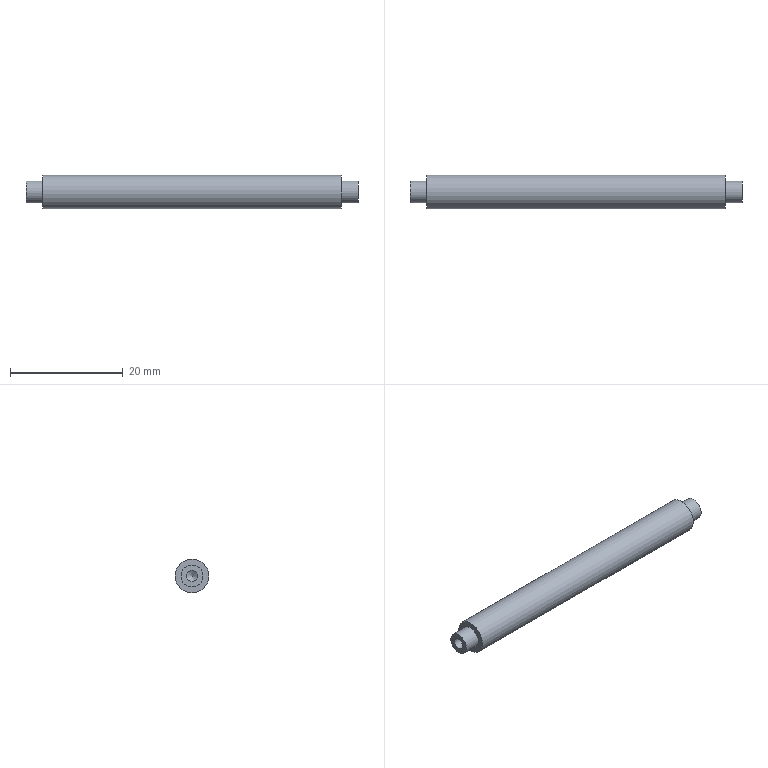Component | NX | SHAFT | 1 solid | 11 faces | box 59 x 6 x 6 mm | volume 1556 mm3 | cylinder 5 | plane 4 | cone 2 | commonest cylinder face diameters 3.9 x2 2 x2 6 x1
STEP:
#1=CARTESIAN_POINT('',(0.,0.,0.));
#2=DIRECTION('',(0.,0.,1.));
#3=DIRECTION('',(1.,0.,0.));
#4=AXIS2_PLACEMENT_3D('',#1,#2,#3);
#5=CARTESIAN_POINT('',(12.144,27.69,-75.915));
#6=VERTEX_POINT('',#5);
#7=CARTESIAN_POINT('',(12.144,27.69,-72.915));
#8=DIRECTION('',(1.,0.,0.));
#9=DIRECTION('',(0.,0.,-1.));
#10=AXIS2_PLACEMENT_3D('',#7,#8,#9);
#11=CIRCLE('',#10,3.);
#12=CARTESIAN_POINT('',(12.144,27.69,-72.915));
#13=DIRECTION('',(-1.,0.,0.));
#14=DIRECTION('',(0.,0.,1.));
#15=AXIS2_PLACEMENT_3D('',#12,#13,#14);
#16=CYLINDRICAL_SURFACE('',#15,3.);
#17=CARTESIAN_POINT('',(9.425,0.));
#18=DIRECTION('',(-1.,0.));
#19=VECTOR('',#18,1.);
#20=LINE('',#17,#19);
#21=(GEOMETRIC_REPRESENTATION_CONTEXT(2)PARAMETRIC_REPRESENTATION_CONTEXT()REPRESENTATION_CONTEXT('',''));
#22=DEFINITIONAL_REPRESENTATION('',(#20),#21);
#23=PCURVE('',#16,#22);
#24=CARTESIAN_POINT('',(12.144,27.69,-72.915));
#25=DIRECTION('',(1.,0.,0.));
#26=DIRECTION('',(0.,0.,-1.));
#27=AXIS2_PLACEMENT_3D('',#24,#25,#26);
#28=PLANE('',#27);
#29=CARTESIAN_POINT('',(0.,0.));
#30=DIRECTION('',(1.,0.));
#31=AXIS2_PLACEMENT_2D('',#29,#30);
#32=CIRCLE('',#31,3.);
#33=(GEOMETRIC_REPRESENTATION_CONTEXT(2)PARAMETRIC_REPRESENTATION_CONTEXT()REPRESENTATION_CONTEXT('',''));
#34=DEFINITIONAL_REPRESENTATION('',(#32),#33);
#35=PCURVE('',#28,#34);
#36=SURFACE_CURVE('',#11,(#23,#35),.PCURVE_S1.);
#37=EDGE_CURVE('',#6,#6,#36,.T.);
#38=ORIENTED_EDGE('',*,*,#37,.F.);
#39=CARTESIAN_POINT('',(-40.856,27.69,-75.915));
#40=VERTEX_POINT('',#39);
#41=CARTESIAN_POINT('',(12.144,27.69,-75.915));
#42=CARTESIAN_POINT('',(-40.856,27.69,-75.915));
#43=B_SPLINE_CURVE_WITH_KNOTS('',1,(#41,#42),.UNSPECIFIED.,.F.,.F.,(2,2),(0.,53.),.PIECEWISE_BEZIER_KNOTS.);
#44=CARTESIAN_POINT('',(9.425,0.));
#45=DIRECTION('',(0.,1.));
#46=VECTOR('',#45,1.);
#47=LINE('',#44,#46);
#48=(GEOMETRIC_REPRESENTATION_CONTEXT(2)PARAMETRIC_REPRESENTATION_CONTEXT()REPRESENTATION_CONTEXT('',''));
#49=DEFINITIONAL_REPRESENTATION('',(#47),#48);
#50=PCURVE('',#16,#49);
#51=CARTESIAN_POINT('',(3.142,0.));
#52=DIRECTION('',(0.,1.));
#53=VECTOR('',#52,1.);
#54=LINE('',#51,#53);
#55=(GEOMETRIC_REPRESENTATION_CONTEXT(2)PARAMETRIC_REPRESENTATION_CONTEXT()REPRESENTATION_CONTEXT('',''));
#56=DEFINITIONAL_REPRESENTATION('',(#54),#55);
#57=PCURVE('',#16,#56);
#58=SEAM_CURVE('',#43,(#50,#57),.PCURVE_S1.);
#59=EDGE_CURVE('',#6,#40,#58,.T.);
#60=ORIENTED_EDGE('',*,*,#59,.T.);
#61=CARTESIAN_POINT('',(-40.856,27.69,-72.915));
#62=DIRECTION('',(1.,0.,0.));
#63=DIRECTION('',(0.,0.,-1.));
#64=AXIS2_PLACEMENT_3D('',#61,#62,#63);
#65=CIRCLE('',#64,3.);
#66=CARTESIAN_POINT('',(9.425,53.));
#67=DIRECTION('',(-1.,0.));
#68=VECTOR('',#67,1.);
#69=LINE('',#66,#68);
#70=(GEOMETRIC_REPRESENTATION_CONTEXT(2)PARAMETRIC_REPRESENTATION_CONTEXT()REPRESENTATION_CONTEXT('',''));
#71=DEFINITIONAL_REPRESENTATION('',(#69),#70);
#72=PCURVE('',#16,#71);
#73=CARTESIAN_POINT('',(-40.856,27.69,-72.915));
#74=DIRECTION('',(1.,0.,0.));
#75=DIRECTION('',(0.,0.,-1.));
#76=AXIS2_PLACEMENT_3D('',#73,#74,#75);
#77=PLANE('',#76);
#78=CARTESIAN_POINT('',(0.,0.));
#79=DIRECTION('',(1.,0.));
#80=AXIS2_PLACEMENT_2D('',#78,#79);
#81=CIRCLE('',#80,3.);
#82=(GEOMETRIC_REPRESENTATION_CONTEXT(2)PARAMETRIC_REPRESENTATION_CONTEXT()REPRESENTATION_CONTEXT('',''));
#83=DEFINITIONAL_REPRESENTATION('',(#81),#82);
#84=PCURVE('',#77,#83);
#85=SURFACE_CURVE('',#65,(#72,#84),.PCURVE_S1.);
#86=EDGE_CURVE('',#40,#40,#85,.T.);
#87=ORIENTED_EDGE('',*,*,#86,.T.);
#88=ORIENTED_EDGE('',*,*,#59,.F.);
#89=EDGE_LOOP('',(#38,#60,#87,#88));
#90=FACE_BOUND('',#89,.T.);
#91=ADVANCED_FACE('',(#90),#16,.T.);
#92=CARTESIAN_POINT('',(12.144,27.69,-74.865));
#93=VERTEX_POINT('',#92);
#94=CARTESIAN_POINT('',(12.144,27.69,-72.915));
#95=DIRECTION('',(1.,0.,0.));
#96=DIRECTION('',(0.,0.,-1.));
#97=AXIS2_PLACEMENT_3D('',#94,#95,#96);
#98=CIRCLE('',#97,1.95);
#99=CARTESIAN_POINT('',(0.,0.));
#100=DIRECTION('',(1.,0.));
#101=AXIS2_PLACEMENT_2D('',#99,#100);
#102=CIRCLE('',#101,1.95);
#103=(GEOMETRIC_REPRESENTATION_CONTEXT(2)PARAMETRIC_REPRESENTATION_CONTEXT()REPRESENTATION_CONTEXT('',''));
#104=DEFINITIONAL_REPRESENTATION('',(#102),#103);
#105=PCURVE('',#28,#104);
#106=CARTESIAN_POINT('',(15.144,27.69,-72.915));
#107=DIRECTION('',(-1.,0.,0.));
#108=DIRECTION('',(0.,0.,1.));
#109=AXIS2_PLACEMENT_3D('',#106,#107,#108);
#110=CYLINDRICAL_SURFACE('',#109,1.95);
#111=CARTESIAN_POINT('',(9.425,3.));
#112=DIRECTION('',(-1.,0.));
#113=VECTOR('',#112,1.);
#114=LINE('',#111,#113);
#115=(GEOMETRIC_REPRESENTATION_CONTEXT(2)PARAMETRIC_REPRESENTATION_CONTEXT()REPRESENTATION_CONTEXT('',''));
#116=DEFINITIONAL_REPRESENTATION('',(#114),#115);
#117=PCURVE('',#110,#116);
#118=SURFACE_CURVE('',#98,(#105,#117),.PCURVE_S1.);
#119=EDGE_CURVE('',#93,#93,#118,.T.);
#120=ORIENTED_EDGE('',*,*,#119,.F.);
#121=EDGE_LOOP('',(#120));
#122=FACE_BOUND('',#121,.T.);
#123=ORIENTED_EDGE('',*,*,#37,.T.);
#124=EDGE_LOOP('',(#123));
#125=FACE_BOUND('',#124,.T.);
#126=ADVANCED_FACE('',(#122,#125),#28,.T.);
#127=CARTESIAN_POINT('',(-40.856,27.69,-74.865));
#128=VERTEX_POINT('',#127);
#129=CARTESIAN_POINT('',(-40.856,27.69,-72.915));
#130=DIRECTION('',(-1.,0.,0.));
#131=DIRECTION('',(0.,0.,-1.));
#132=AXIS2_PLACEMENT_3D('',#129,#130,#131);
#133=CIRCLE('',#132,1.95);
#134=CARTESIAN_POINT('',(1.95,0.));
#135=CARTESIAN_POINT('',(1.95,-3.377));
#136=CARTESIAN_POINT('',(-0.975,-1.689));
#137=CARTESIAN_POINT('',(-3.9,-0.));
#138=CARTESIAN_POINT('',(-0.975,1.689));
#139=CARTESIAN_POINT('',(1.95,3.377));
#140=CARTESIAN_POINT('',(1.95,0.));
#141=(BOUNDED_CURVE()B_SPLINE_CURVE(2,(#134,#135,#136,#137,#138,#139,#140),.UNSPECIFIED.,.T.,.F.)B_SPLINE_CURVE_WITH_KNOTS((1,2,2,2,2,1),(-2.094,0.,2.094,4.189,6.283,8.378),.UNSPECIFIED.)CURVE()GEOMETRIC_REPRESENTATION_ITEM()RATIONAL_B_SPLINE_CURVE((1.,0.5,1.,0.5,1.,0.5,1.))REPRESENTATION_ITEM(''));
#142=(GEOMETRIC_REPRESENTATION_CONTEXT(2)PARAMETRIC_REPRESENTATION_CONTEXT()REPRESENTATION_CONTEXT('',''));
#143=DEFINITIONAL_REPRESENTATION('',(#141),#142);
#144=PCURVE('',#77,#143);
#145=CARTESIAN_POINT('',(-43.856,27.69,-72.915));
#146=DIRECTION('',(1.,0.,0.));
#147=DIRECTION('',(0.,0.,-1.));
#148=AXIS2_PLACEMENT_3D('',#145,#146,#147);
#149=CYLINDRICAL_SURFACE('',#148,1.95);
#150=CARTESIAN_POINT('',(6.283,3.));
#151=DIRECTION('',(-1.,0.));
#152=VECTOR('',#151,1.);
#153=LINE('',#150,#152);
#154=(GEOMETRIC_REPRESENTATION_CONTEXT(2)PARAMETRIC_REPRESENTATION_CONTEXT()REPRESENTATION_CONTEXT('',''));
#155=DEFINITIONAL_REPRESENTATION('',(#153),#154);
#156=PCURVE('',#149,#155);
#157=SURFACE_CURVE('',#133,(#144,#156),.PCURVE_S1.);
#158=EDGE_CURVE('',#128,#128,#157,.T.);
#159=ORIENTED_EDGE('',*,*,#158,.F.);
#160=EDGE_LOOP('',(#159));
#161=FACE_BOUND('',#160,.T.);
#162=ORIENTED_EDGE('',*,*,#86,.F.);
#163=EDGE_LOOP('',(#162));
#164=FACE_BOUND('',#163,.T.);
#165=ADVANCED_FACE('',(#161,#164),#77,.F.);
#166=CARTESIAN_POINT('',(15.144,27.69,-74.865));
#167=VERTEX_POINT('',#166);
#168=CARTESIAN_POINT('',(15.144,27.69,-72.915));
#169=DIRECTION('',(1.,0.,0.));
#170=DIRECTION('',(0.,0.,-1.));
#171=AXIS2_PLACEMENT_3D('',#168,#169,#170);
#172=CIRCLE('',#171,1.95);
#173=CARTESIAN_POINT('',(9.425,0.));
#174=DIRECTION('',(-1.,0.));
#175=VECTOR('',#174,1.);
#176=LINE('',#173,#175);
#177=(GEOMETRIC_REPRESENTATION_CONTEXT(2)PARAMETRIC_REPRESENTATION_CONTEXT()REPRESENTATION_CONTEXT('',''));
#178=DEFINITIONAL_REPRESENTATION('',(#176),#177);
#179=PCURVE('',#110,#178);
#180=CARTESIAN_POINT('',(15.144,27.69,-72.915));
#181=DIRECTION('',(1.,0.,0.));
#182=DIRECTION('',(0.,0.,-1.));
#183=AXIS2_PLACEMENT_3D('',#180,#181,#182);
#184=PLANE('',#183);
#185=CARTESIAN_POINT('',(0.,0.));
#186=DIRECTION('',(1.,0.));
#187=AXIS2_PLACEMENT_2D('',#185,#186);
#188=CIRCLE('',#187,1.95);
#189=(GEOMETRIC_REPRESENTATION_CONTEXT(2)PARAMETRIC_REPRESENTATION_CONTEXT()REPRESENTATION_CONTEXT('',''));
#190=DEFINITIONAL_REPRESENTATION('',(#188),#189);
#191=PCURVE('',#184,#190);
#192=SURFACE_CURVE('',#172,(#179,#191),.PCURVE_S1.);
#193=EDGE_CURVE('',#167,#167,#192,.T.);
#194=ORIENTED_EDGE('',*,*,#193,.F.);
#195=CARTESIAN_POINT('',(15.144,27.69,-74.865));
#196=CARTESIAN_POINT('',(12.144,27.69,-74.865));
#197=B_SPLINE_CURVE_WITH_KNOTS('',1,(#195,#196),.UNSPECIFIED.,.F.,.F.,(2,2),(0.,3.),.PIECEWISE_BEZIER_KNOTS.);
#198=CARTESIAN_POINT('',(9.425,0.));
#199=DIRECTION('',(0.,1.));
#200=VECTOR('',#199,1.);
#201=LINE('',#198,#200);
#202=(GEOMETRIC_REPRESENTATION_CONTEXT(2)PARAMETRIC_REPRESENTATION_CONTEXT()REPRESENTATION_CONTEXT('',''));
#203=DEFINITIONAL_REPRESENTATION('',(#201),#202);
#204=PCURVE('',#110,#203);
#205=CARTESIAN_POINT('',(3.142,0.));
#206=DIRECTION('',(0.,1.));
#207=VECTOR('',#206,1.);
#208=LINE('',#205,#207);
#209=(GEOMETRIC_REPRESENTATION_CONTEXT(2)PARAMETRIC_REPRESENTATION_CONTEXT()REPRESENTATION_CONTEXT('',''));
#210=DEFINITIONAL_REPRESENTATION('',(#208),#209);
#211=PCURVE('',#110,#210);
#212=SEAM_CURVE('',#197,(#204,#211),.PCURVE_S1.);
#213=EDGE_CURVE('',#167,#93,#212,.T.);
#214=ORIENTED_EDGE('',*,*,#213,.T.);
#215=ORIENTED_EDGE('',*,*,#119,.T.);
#216=ORIENTED_EDGE('',*,*,#213,.F.);
#217=EDGE_LOOP('',(#194,#214,#215,#216));
#218=FACE_BOUND('',#217,.T.);
#219=ADVANCED_FACE('',(#218),#110,.T.);
#220=CARTESIAN_POINT('',(15.144,27.69,-71.915));
#221=VERTEX_POINT('',#220);
#222=CARTESIAN_POINT('',(15.144,27.69,-72.915));
#223=DIRECTION('',(-1.,0.,0.));
#224=DIRECTION('',(0.,0.,1.));
#225=AXIS2_PLACEMENT_3D('',#222,#223,#224);
#226=CIRCLE('',#225,1.);
#227=CARTESIAN_POINT('',(-1.,0.));
#228=CARTESIAN_POINT('',(-1.,1.732));
#229=CARTESIAN_POINT('',(0.5,0.866));
#230=CARTESIAN_POINT('',(2.,0.));
#231=CARTESIAN_POINT('',(0.5,-0.866));
#232=CARTESIAN_POINT('',(-1.,-1.732));
#233=CARTESIAN_POINT('',(-1.,0.));
#234=(BOUNDED_CURVE()B_SPLINE_CURVE(2,(#227,#228,#229,#230,#231,#232,#233),.UNSPECIFIED.,.T.,.F.)B_SPLINE_CURVE_WITH_KNOTS((1,2,2,2,2,1),(-2.094,0.,2.094,4.189,6.283,8.378),.UNSPECIFIED.)CURVE()GEOMETRIC_REPRESENTATION_ITEM()RATIONAL_B_SPLINE_CURVE((1.,0.5,1.,0.5,1.,0.5,1.))REPRESENTATION_ITEM(''));
#235=(GEOMETRIC_REPRESENTATION_CONTEXT(2)PARAMETRIC_REPRESENTATION_CONTEXT()REPRESENTATION_CONTEXT('',''));
#236=DEFINITIONAL_REPRESENTATION('',(#234),#235);
#237=PCURVE('',#184,#236);
#238=CARTESIAN_POINT('',(15.144,27.69,-72.915));
#239=DIRECTION('',(-1.,0.,0.));
#240=DIRECTION('',(0.,0.,1.));
#241=AXIS2_PLACEMENT_3D('',#238,#239,#240);
#242=CYLINDRICAL_SURFACE('',#241,1.);
#243=CARTESIAN_POINT('',(0.,0.));
#244=DIRECTION('',(1.,0.));
#245=VECTOR('',#244,1.);
#246=LINE('',#243,#245);
#247=(GEOMETRIC_REPRESENTATION_CONTEXT(2)PARAMETRIC_REPRESENTATION_CONTEXT()REPRESENTATION_CONTEXT('',''));
#248=DEFINITIONAL_REPRESENTATION('',(#246),#247);
#249=PCURVE('',#242,#248);
#250=SURFACE_CURVE('',#226,(#237,#249),.PCURVE_S1.);
#251=EDGE_CURVE('',#221,#221,#250,.T.);
#252=ORIENTED_EDGE('',*,*,#251,.T.);
#253=EDGE_LOOP('',(#252));
#254=FACE_BOUND('',#253,.T.);
#255=ORIENTED_EDGE('',*,*,#193,.T.);
#256=EDGE_LOOP('',(#255));
#257=FACE_BOUND('',#256,.T.);
#258=ADVANCED_FACE('',(#254,#257),#184,.T.);
#259=CARTESIAN_POINT('',(-43.856,27.69,-74.865));
#260=VERTEX_POINT('',#259);
#261=CARTESIAN_POINT('',(-43.856,27.69,-72.915));
#262=DIRECTION('',(-1.,0.,0.));
#263=DIRECTION('',(0.,0.,-1.));
#264=AXIS2_PLACEMENT_3D('',#261,#262,#263);
#265=CIRCLE('',#264,1.95);
#266=CARTESIAN_POINT('',(6.283,0.));
#267=DIRECTION('',(-1.,0.));
#268=VECTOR('',#267,1.);
#269=LINE('',#266,#268);
#270=(GEOMETRIC_REPRESENTATION_CONTEXT(2)PARAMETRIC_REPRESENTATION_CONTEXT()REPRESENTATION_CONTEXT('',''));
#271=DEFINITIONAL_REPRESENTATION('',(#269),#270);
#272=PCURVE('',#149,#271);
#273=CARTESIAN_POINT('',(-43.856,27.69,-72.915));
#274=DIRECTION('',(-1.,0.,0.));
#275=DIRECTION('',(0.,0.,1.));
#276=AXIS2_PLACEMENT_3D('',#273,#274,#275);
#277=PLANE('',#276);
#278=CARTESIAN_POINT('',(0.,0.));
#279=DIRECTION('',(-1.,0.));
#280=AXIS2_PLACEMENT_2D('',#278,#279);
#281=CIRCLE('',#280,1.95);
#282=(GEOMETRIC_REPRESENTATION_CONTEXT(2)PARAMETRIC_REPRESENTATION_CONTEXT()REPRESENTATION_CONTEXT('',''));
#283=DEFINITIONAL_REPRESENTATION('',(#281),#282);
#284=PCURVE('',#277,#283);
#285=SURFACE_CURVE('',#265,(#272,#284),.PCURVE_S1.);
#286=EDGE_CURVE('',#260,#260,#285,.T.);
#287=ORIENTED_EDGE('',*,*,#286,.F.);
#288=CARTESIAN_POINT('',(-43.856,27.69,-74.865));
#289=CARTESIAN_POINT('',(-40.856,27.69,-74.865));
#290=B_SPLINE_CURVE_WITH_KNOTS('',1,(#288,#289),.UNSPECIFIED.,.F.,.F.,(2,2),(0.,3.),.PIECEWISE_BEZIER_KNOTS.);
#291=CARTESIAN_POINT('',(6.283,0.));
#292=DIRECTION('',(0.,1.));
#293=VECTOR('',#292,1.);
#294=LINE('',#291,#293);
#295=(GEOMETRIC_REPRESENTATION_CONTEXT(2)PARAMETRIC_REPRESENTATION_CONTEXT()REPRESENTATION_CONTEXT('',''));
#296=DEFINITIONAL_REPRESENTATION('',(#294),#295);
#297=PCURVE('',#149,#296);
#298=CARTESIAN_POINT('',(0.,0.));
#299=DIRECTION('',(0.,1.));
#300=VECTOR('',#299,1.);
#301=LINE('',#298,#300);
#302=(GEOMETRIC_REPRESENTATION_CONTEXT(2)PARAMETRIC_REPRESENTATION_CONTEXT()REPRESENTATION_CONTEXT('',''));
#303=DEFINITIONAL_REPRESENTATION('',(#301),#302);
#304=PCURVE('',#149,#303);
#305=SEAM_CURVE('',#290,(#297,#304),.PCURVE_S1.);
#306=EDGE_CURVE('',#260,#128,#305,.T.);
#307=ORIENTED_EDGE('',*,*,#306,.T.);
#308=ORIENTED_EDGE('',*,*,#158,.T.);
#309=ORIENTED_EDGE('',*,*,#306,.F.);
#310=EDGE_LOOP('',(#287,#307,#308,#309));
#311=FACE_BOUND('',#310,.T.);
#312=ADVANCED_FACE('',(#311),#149,.T.);
#313=CARTESIAN_POINT('',(-43.856,27.69,-73.915));
#314=VERTEX_POINT('',#313);
#315=CARTESIAN_POINT('',(-43.856,27.69,-72.915));
#316=DIRECTION('',(1.,0.,0.));
#317=DIRECTION('',(0.,0.,-1.));
#318=AXIS2_PLACEMENT_3D('',#315,#316,#317);
#319=CIRCLE('',#318,1.);
#320=CARTESIAN_POINT('',(-1.,0.));
#321=CARTESIAN_POINT('',(-1.,1.732));
#322=CARTESIAN_POINT('',(0.5,0.866));
#323=CARTESIAN_POINT('',(2.,0.));
#324=CARTESIAN_POINT('',(0.5,-0.866));
#325=CARTESIAN_POINT('',(-1.,-1.732));
#326=CARTESIAN_POINT('',(-1.,0.));
#327=(BOUNDED_CURVE()B_SPLINE_CURVE(2,(#320,#321,#322,#323,#324,#325,#326),.UNSPECIFIED.,.T.,.F.)B_SPLINE_CURVE_WITH_KNOTS((1,2,2,2,2,1),(-2.094,0.,2.094,4.189,6.283,8.378),.UNSPECIFIED.)CURVE()GEOMETRIC_REPRESENTATION_ITEM()RATIONAL_B_SPLINE_CURVE((1.,0.5,1.,0.5,1.,0.5,1.))REPRESENTATION_ITEM(''));
#328=(GEOMETRIC_REPRESENTATION_CONTEXT(2)PARAMETRIC_REPRESENTATION_CONTEXT()REPRESENTATION_CONTEXT('',''));
#329=DEFINITIONAL_REPRESENTATION('',(#327),#328);
#330=PCURVE('',#277,#329);
#331=CARTESIAN_POINT('',(-43.856,27.69,-72.915));
#332=DIRECTION('',(1.,0.,0.));
#333=DIRECTION('',(0.,0.,-1.));
#334=AXIS2_PLACEMENT_3D('',#331,#332,#333);
#335=CYLINDRICAL_SURFACE('',#334,1.);
#336=CARTESIAN_POINT('',(0.,0.));
#337=DIRECTION('',(1.,0.));
#338=VECTOR('',#337,1.);
#339=LINE('',#336,#338);
#340=(GEOMETRIC_REPRESENTATION_CONTEXT(2)PARAMETRIC_REPRESENTATION_CONTEXT()REPRESENTATION_CONTEXT('',''));
#341=DEFINITIONAL_REPRESENTATION('',(#339),#340);
#342=PCURVE('',#335,#341);
#343=SURFACE_CURVE('',#319,(#330,#342),.PCURVE_S1.);
#344=EDGE_CURVE('',#314,#314,#343,.T.);
#345=ORIENTED_EDGE('',*,*,#344,.T.);
#346=EDGE_LOOP('',(#345));
#347=FACE_BOUND('',#346,.T.);
#348=ORIENTED_EDGE('',*,*,#286,.T.);
#349=EDGE_LOOP('',(#348));
#350=FACE_BOUND('',#349,.T.);
#351=ADVANCED_FACE('',(#347,#350),#277,.T.);
#352=CARTESIAN_POINT('',(-41.856,27.69,-71.915));
#353=VERTEX_POINT('',#352);
#354=CARTESIAN_POINT('',(-41.856,27.69,-73.915));
#355=VERTEX_POINT('',#354);
#356=CARTESIAN_POINT('',(-41.856,27.69,-72.915));
#357=DIRECTION('',(-1.,0.,0.));
#358=DIRECTION('',(0.,0.,-1.));
#359=AXIS2_PLACEMENT_3D('',#356,#357,#358);
#360=CIRCLE('',#359,1.);
#361=CARTESIAN_POINT('',(-41.856,27.69,-72.915));
#362=DIRECTION('',(-1.,0.,0.));
#363=DIRECTION('',(0.,0.,1.));
#364=AXIS2_PLACEMENT_3D('',#361,#362,#363);
#365=CONICAL_SURFACE('',#364,1.,1.03);
#366=CARTESIAN_POINT('',(-3.142,0.));
#367=DIRECTION('',(1.,0.));
#368=VECTOR('',#367,1.);
#369=LINE('',#366,#368);
#370=(GEOMETRIC_REPRESENTATION_CONTEXT(2)PARAMETRIC_REPRESENTATION_CONTEXT()REPRESENTATION_CONTEXT('',''));
#371=DEFINITIONAL_REPRESENTATION('',(#369),#370);
#372=PCURVE('',#365,#371);
#373=CARTESIAN_POINT('',(6.283,2.));
#374=DIRECTION('',(-1.,0.));
#375=VECTOR('',#374,1.);
#376=LINE('',#373,#375);
#377=(GEOMETRIC_REPRESENTATION_CONTEXT(2)PARAMETRIC_REPRESENTATION_CONTEXT()REPRESENTATION_CONTEXT('',''));
#378=DEFINITIONAL_REPRESENTATION('',(#376),#377);
#379=PCURVE('',#335,#378);
#380=SURFACE_CURVE('',#360,(#372,#379),.PCURVE_S1.);
#381=EDGE_CURVE('',#353,#355,#380,.T.);
#382=ORIENTED_EDGE('',*,*,#381,.F.);
#383=CARTESIAN_POINT('',(-41.255,27.69,-72.915));
#384=VERTEX_POINT('',#383);
#385=CARTESIAN_POINT('',(-41.255,27.69,-72.915));
#386=CARTESIAN_POINT('',(-41.856,27.69,-71.915));
#387=B_SPLINE_CURVE_WITH_KNOTS('',1,(#385,#386),.UNSPECIFIED.,.F.,.F.,(2,2),(-1.167,0.),.PIECEWISE_BEZIER_KNOTS.);
#388=CARTESIAN_POINT('',(0.,0.));
#389=DIRECTION('',(0.,1.));
#390=VECTOR('',#389,1.);
#391=LINE('',#388,#390);
#392=(GEOMETRIC_REPRESENTATION_CONTEXT(2)PARAMETRIC_REPRESENTATION_CONTEXT()REPRESENTATION_CONTEXT('',''));
#393=DEFINITIONAL_REPRESENTATION('',(#391),#392);
#394=PCURVE('',#365,#393);
#395=CARTESIAN_POINT('',(6.283,0.));
#396=DIRECTION('',(0.,1.));
#397=VECTOR('',#396,1.);
#398=LINE('',#395,#397);
#399=(GEOMETRIC_REPRESENTATION_CONTEXT(2)PARAMETRIC_REPRESENTATION_CONTEXT()REPRESENTATION_CONTEXT('',''));
#400=DEFINITIONAL_REPRESENTATION('',(#398),#399);
#401=PCURVE('',#365,#400);
#402=SEAM_CURVE('',#387,(#394,#401),.PCURVE_S1.);
#403=EDGE_CURVE('',#384,#353,#402,.T.);
#404=ORIENTED_EDGE('',*,*,#403,.F.);
#405=ORIENTED_EDGE('',*,*,#403,.T.);
#406=CARTESIAN_POINT('',(-41.856,27.69,-72.915));
#407=DIRECTION('',(-1.,0.,0.));
#408=DIRECTION('',(0.,0.,-1.));
#409=AXIS2_PLACEMENT_3D('',#406,#407,#408);
#410=CIRCLE('',#409,1.);
#411=CARTESIAN_POINT('',(3.142,0.));
#412=DIRECTION('',(1.,0.));
#413=VECTOR('',#412,1.);
#414=LINE('',#411,#413);
#415=(GEOMETRIC_REPRESENTATION_CONTEXT(2)PARAMETRIC_REPRESENTATION_CONTEXT()REPRESENTATION_CONTEXT('',''));
#416=DEFINITIONAL_REPRESENTATION('',(#414),#415);
#417=PCURVE('',#365,#416);
#418=CARTESIAN_POINT('',(6.283,2.));
#419=DIRECTION('',(-1.,0.));
#420=VECTOR('',#419,1.);
#421=LINE('',#418,#420);
#422=(GEOMETRIC_REPRESENTATION_CONTEXT(2)PARAMETRIC_REPRESENTATION_CONTEXT()REPRESENTATION_CONTEXT('',''));
#423=DEFINITIONAL_REPRESENTATION('',(#421),#422);
#424=PCURVE('',#335,#423);
#425=SURFACE_CURVE('',#410,(#417,#424),.PCURVE_S1.);
#426=EDGE_CURVE('',#355,#353,#425,.T.);
#427=ORIENTED_EDGE('',*,*,#426,.F.);
#428=EDGE_LOOP('',(#382,#404,#405,#427));
#429=FACE_BOUND('',#428,.F.);
#430=ADVANCED_FACE('',(#429),#365,.F.);
#431=ORIENTED_EDGE('',*,*,#381,.T.);
#432=CARTESIAN_POINT('',(-43.856,27.69,-73.915));
#433=CARTESIAN_POINT('',(-41.856,27.69,-73.915));
#434=B_SPLINE_CURVE_WITH_KNOTS('',1,(#432,#433),.UNSPECIFIED.,.F.,.F.,(2,2),(0.,2.),.PIECEWISE_BEZIER_KNOTS.);
#435=CARTESIAN_POINT('',(0.,0.));
#436=DIRECTION('',(0.,1.));
#437=VECTOR('',#436,1.);
#438=LINE('',#435,#437);
#439=(GEOMETRIC_REPRESENTATION_CONTEXT(2)PARAMETRIC_REPRESENTATION_CONTEXT()REPRESENTATION_CONTEXT('',''));
#440=DEFINITIONAL_REPRESENTATION('',(#438),#439);
#441=PCURVE('',#335,#440);
#442=CARTESIAN_POINT('',(6.283,0.));
#443=DIRECTION('',(0.,1.));
#444=VECTOR('',#443,1.);
#445=LINE('',#442,#444);
#446=(GEOMETRIC_REPRESENTATION_CONTEXT(2)PARAMETRIC_REPRESENTATION_CONTEXT()REPRESENTATION_CONTEXT('',''));
#447=DEFINITIONAL_REPRESENTATION('',(#445),#446);
#448=PCURVE('',#335,#447);
#449=SEAM_CURVE('',#434,(#441,#448),.PCURVE_S1.);
#450=EDGE_CURVE('',#314,#355,#449,.T.);
#451=ORIENTED_EDGE('',*,*,#450,.F.);
#452=ORIENTED_EDGE('',*,*,#344,.T.);
#453=ORIENTED_EDGE('',*,*,#450,.T.);
#454=ORIENTED_EDGE('',*,*,#426,.T.);
#455=EDGE_LOOP('',(#431,#451,#452,#453,#454));
#456=FACE_BOUND('',#455,.F.);
#457=ADVANCED_FACE('',(#456),#335,.F.);
#458=CARTESIAN_POINT('',(13.144,27.69,-73.915));
#459=VERTEX_POINT('',#458);
#460=CARTESIAN_POINT('',(13.144,27.69,-71.915));
#461=VERTEX_POINT('',#460);
#462=CARTESIAN_POINT('',(13.144,27.69,-72.915));
#463=DIRECTION('',(1.,0.,0.));
#464=DIRECTION('',(0.,0.,1.));
#465=AXIS2_PLACEMENT_3D('',#462,#463,#464);
#466=CIRCLE('',#465,1.);
#467=CARTESIAN_POINT('',(13.144,27.69,-72.915));
#468=DIRECTION('',(1.,0.,0.));
#469=DIRECTION('',(0.,0.,-1.));
#470=AXIS2_PLACEMENT_3D('',#467,#468,#469);
#471=CONICAL_SURFACE('',#470,1.,1.03);
#472=CARTESIAN_POINT('',(-3.142,0.));
#473=DIRECTION('',(1.,0.));
#474=VECTOR('',#473,1.);
#475=LINE('',#472,#474);
#476=(GEOMETRIC_REPRESENTATION_CONTEXT(2)PARAMETRIC_REPRESENTATION_CONTEXT()REPRESENTATION_CONTEXT('',''));
#477=DEFINITIONAL_REPRESENTATION('',(#475),#476);
#478=PCURVE('',#471,#477);
#479=CARTESIAN_POINT('',(6.283,2.));
#480=DIRECTION('',(-1.,0.));
#481=VECTOR('',#480,1.);
#482=LINE('',#479,#481);
#483=(GEOMETRIC_REPRESENTATION_CONTEXT(2)PARAMETRIC_REPRESENTATION_CONTEXT()REPRESENTATION_CONTEXT('',''));
#484=DEFINITIONAL_REPRESENTATION('',(#482),#483);
#485=PCURVE('',#242,#484);
#486=SURFACE_CURVE('',#466,(#478,#485),.PCURVE_S1.);
#487=EDGE_CURVE('',#459,#461,#486,.T.);
#488=ORIENTED_EDGE('',*,*,#487,.F.);
#489=CARTESIAN_POINT('',(12.543,27.69,-72.915));
#490=VERTEX_POINT('',#489);
#491=CARTESIAN_POINT('',(12.543,27.69,-72.915));
#492=CARTESIAN_POINT('',(13.144,27.69,-73.915));
#493=B_SPLINE_CURVE_WITH_KNOTS('',1,(#491,#492),.UNSPECIFIED.,.F.,.F.,(2,2),(-1.167,0.),.PIECEWISE_BEZIER_KNOTS.);
#494=CARTESIAN_POINT('',(0.,0.));
#495=DIRECTION('',(0.,1.));
#496=VECTOR('',#495,1.);
#497=LINE('',#494,#496);
#498=(GEOMETRIC_REPRESENTATION_CONTEXT(2)PARAMETRIC_REPRESENTATION_CONTEXT()REPRESENTATION_CONTEXT('',''));
#499=DEFINITIONAL_REPRESENTATION('',(#497),#498);
#500=PCURVE('',#471,#499);
#501=CARTESIAN_POINT('',(6.283,0.));
#502=DIRECTION('',(0.,1.));
#503=VECTOR('',#502,1.);
#504=LINE('',#501,#503);
#505=(GEOMETRIC_REPRESENTATION_CONTEXT(2)PARAMETRIC_REPRESENTATION_CONTEXT()REPRESENTATION_CONTEXT('',''));
#506=DEFINITIONAL_REPRESENTATION('',(#504),#505);
#507=PCURVE('',#471,#506);
#508=SEAM_CURVE('',#493,(#500,#507),.PCURVE_S1.);
#509=EDGE_CURVE('',#490,#459,#508,.T.);
#510=ORIENTED_EDGE('',*,*,#509,.F.);
#511=ORIENTED_EDGE('',*,*,#509,.T.);
#512=CARTESIAN_POINT('',(13.144,27.69,-72.915));
#513=DIRECTION('',(1.,0.,0.));
#514=DIRECTION('',(0.,0.,1.));
#515=AXIS2_PLACEMENT_3D('',#512,#513,#514);
#516=CIRCLE('',#515,1.);
#517=CARTESIAN_POINT('',(3.142,0.));
#518=DIRECTION('',(1.,0.));
#519=VECTOR('',#518,1.);
#520=LINE('',#517,#519);
#521=(GEOMETRIC_REPRESENTATION_CONTEXT(2)PARAMETRIC_REPRESENTATION_CONTEXT()REPRESENTATION_CONTEXT('',''));
#522=DEFINITIONAL_REPRESENTATION('',(#520),#521);
#523=PCURVE('',#471,#522);
#524=CARTESIAN_POINT('',(6.283,2.));
#525=DIRECTION('',(-1.,0.));
#526=VECTOR('',#525,1.);
#527=LINE('',#524,#526);
#528=(GEOMETRIC_REPRESENTATION_CONTEXT(2)PARAMETRIC_REPRESENTATION_CONTEXT()REPRESENTATION_CONTEXT('',''));
#529=DEFINITIONAL_REPRESENTATION('',(#527),#528);
#530=PCURVE('',#242,#529);
#531=SURFACE_CURVE('',#516,(#523,#530),.PCURVE_S1.);
#532=EDGE_CURVE('',#461,#459,#531,.T.);
#533=ORIENTED_EDGE('',*,*,#532,.F.);
#534=EDGE_LOOP('',(#488,#510,#511,#533));
#535=FACE_BOUND('',#534,.F.);
#536=ADVANCED_FACE('',(#535),#471,.F.);
#537=ORIENTED_EDGE('',*,*,#487,.T.);
#538=CARTESIAN_POINT('',(15.144,27.69,-71.915));
#539=CARTESIAN_POINT('',(13.144,27.69,-71.915));
#540=B_SPLINE_CURVE_WITH_KNOTS('',1,(#538,#539),.UNSPECIFIED.,.F.,.F.,(2,2),(0.,2.),.PIECEWISE_BEZIER_KNOTS.);
#541=CARTESIAN_POINT('',(0.,0.));
#542=DIRECTION('',(0.,1.));
#543=VECTOR('',#542,1.);
#544=LINE('',#541,#543);
#545=(GEOMETRIC_REPRESENTATION_CONTEXT(2)PARAMETRIC_REPRESENTATION_CONTEXT()REPRESENTATION_CONTEXT('',''));
#546=DEFINITIONAL_REPRESENTATION('',(#544),#545);
#547=PCURVE('',#242,#546);
#548=CARTESIAN_POINT('',(6.283,0.));
#549=DIRECTION('',(0.,1.));
#550=VECTOR('',#549,1.);
#551=LINE('',#548,#550);
#552=(GEOMETRIC_REPRESENTATION_CONTEXT(2)PARAMETRIC_REPRESENTATION_CONTEXT()REPRESENTATION_CONTEXT('',''));
#553=DEFINITIONAL_REPRESENTATION('',(#551),#552);
#554=PCURVE('',#242,#553);
#555=SEAM_CURVE('',#540,(#547,#554),.PCURVE_S1.);
#556=EDGE_CURVE('',#221,#461,#555,.T.);
#557=ORIENTED_EDGE('',*,*,#556,.F.);
#558=ORIENTED_EDGE('',*,*,#251,.T.);
#559=ORIENTED_EDGE('',*,*,#556,.T.);
#560=ORIENTED_EDGE('',*,*,#532,.T.);
#561=EDGE_LOOP('',(#537,#557,#558,#559,#560));
#562=FACE_BOUND('',#561,.F.);
#563=ADVANCED_FACE('',(#562),#242,.F.);
#564=CLOSED_SHELL('',(#91,#126,#165,#219,#258,#312,#351,#430,#457,#536,#563));
#565=MANIFOLD_SOLID_BREP('',#564);
#566=(LENGTH_UNIT()NAMED_UNIT(*)SI_UNIT(.MILLI.,.METRE.));
#567=UNCERTAINTY_MEASURE_WITH_UNIT(LENGTH_MEASURE(0.00001),#566,'','');
#568=(NAMED_UNIT(*)PLANE_ANGLE_UNIT()SI_UNIT($,.RADIAN.));
#569=(NAMED_UNIT(*)SI_UNIT($,.STERADIAN.)SOLID_ANGLE_UNIT());
#570=(GEOMETRIC_REPRESENTATION_CONTEXT(3)GLOBAL_UNCERTAINTY_ASSIGNED_CONTEXT((#567))GLOBAL_UNIT_ASSIGNED_CONTEXT((#566,#568,#569))REPRESENTATION_CONTEXT('',''));
#571=ADVANCED_BREP_SHAPE_REPRESENTATION('',(#4,#565),#570);